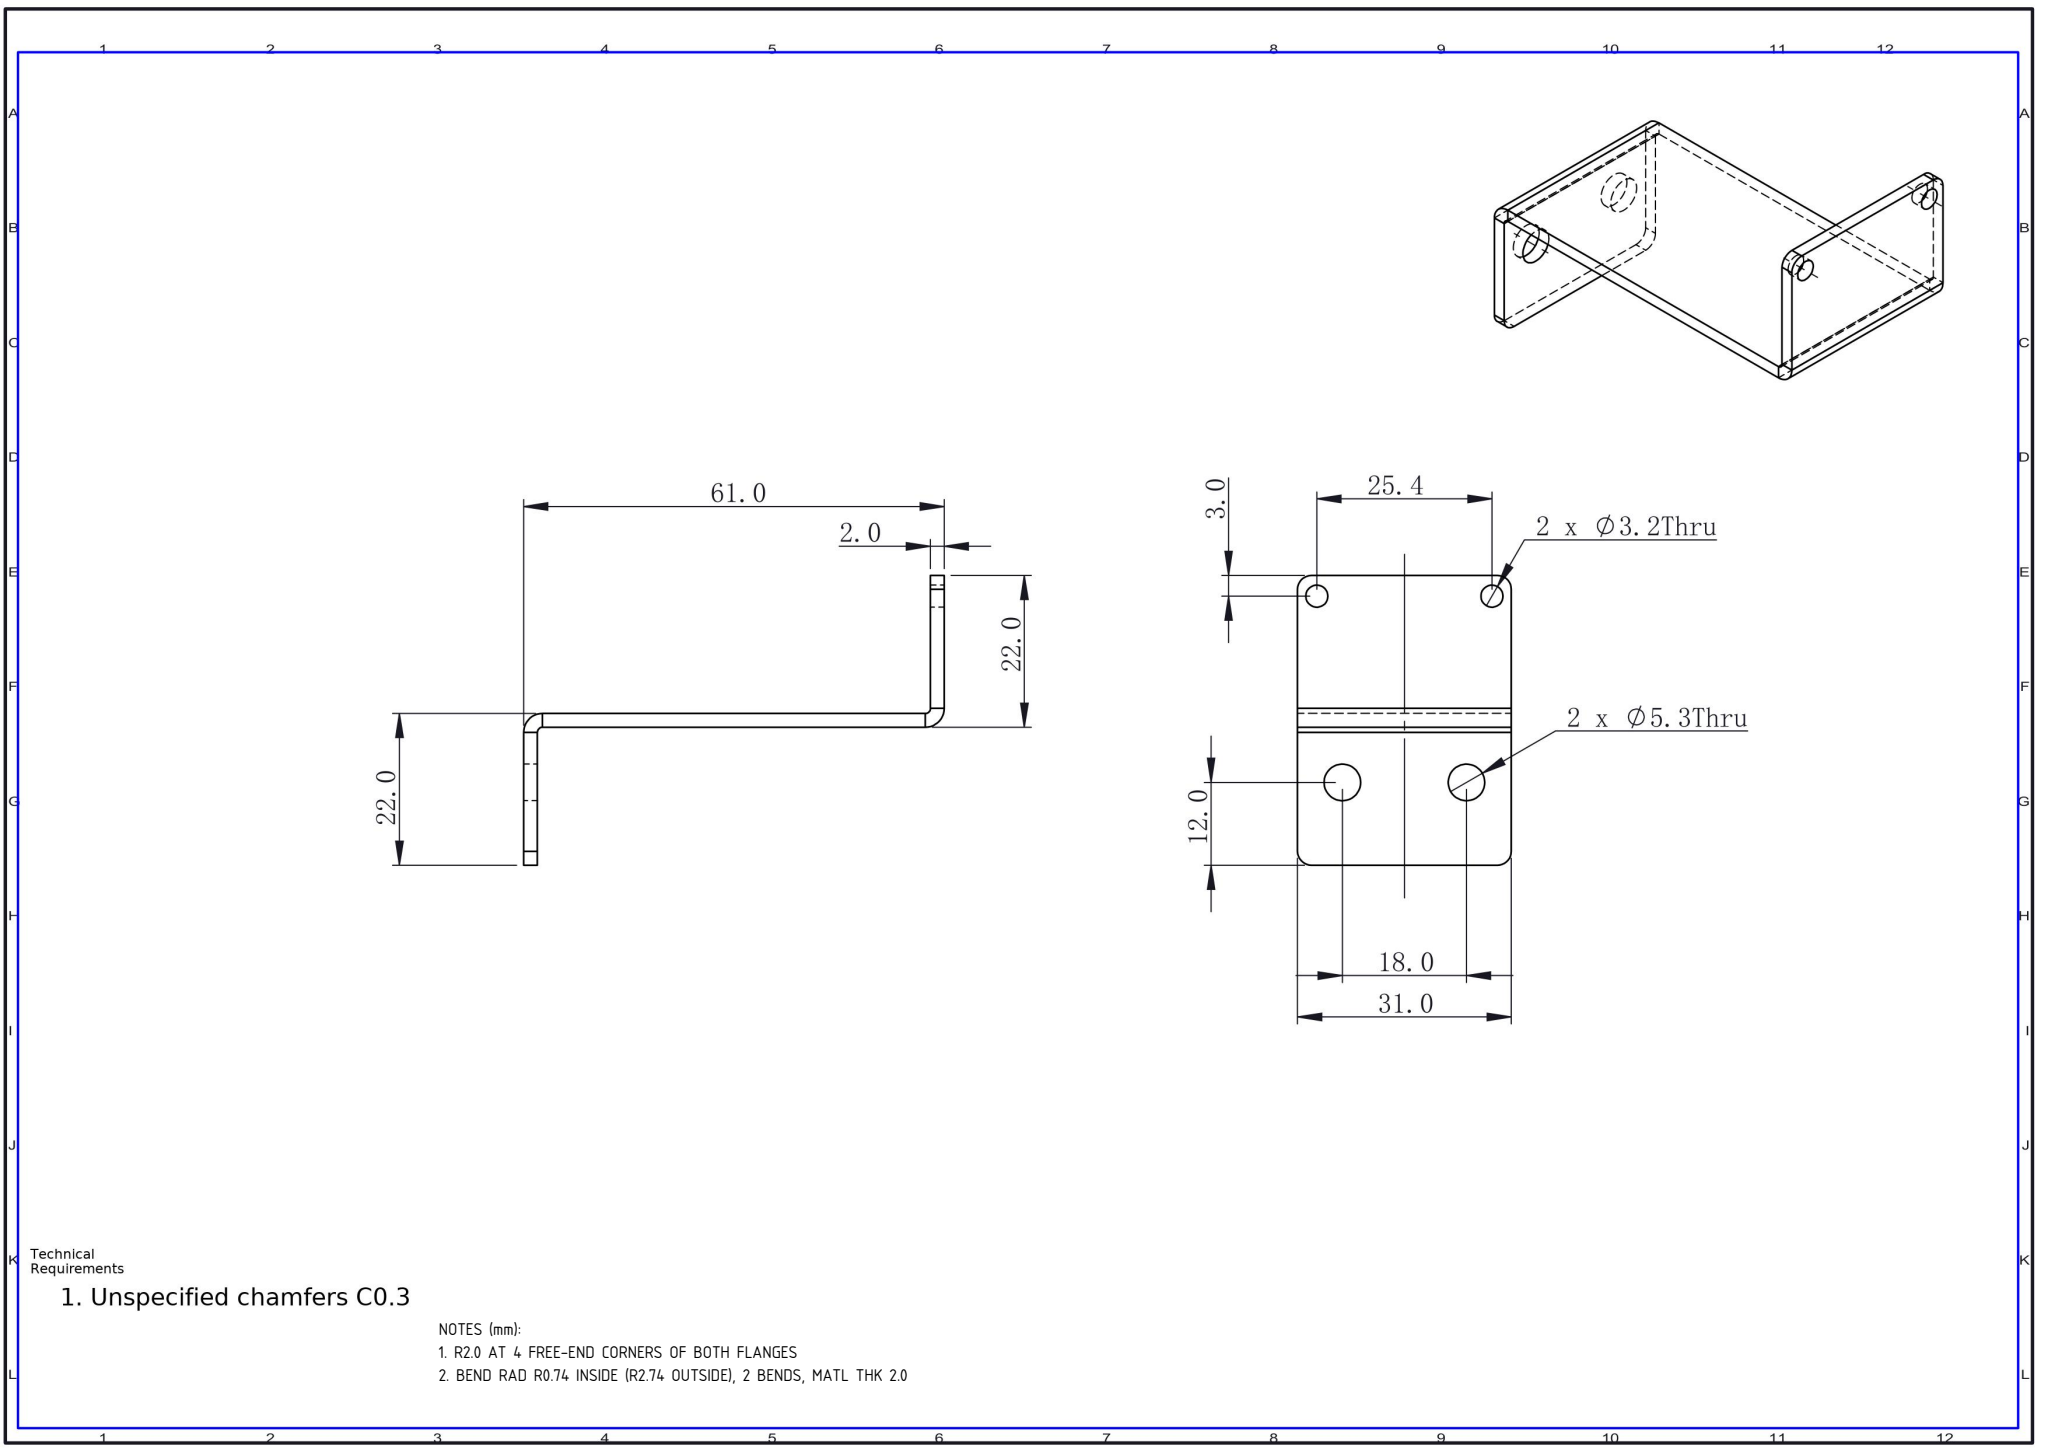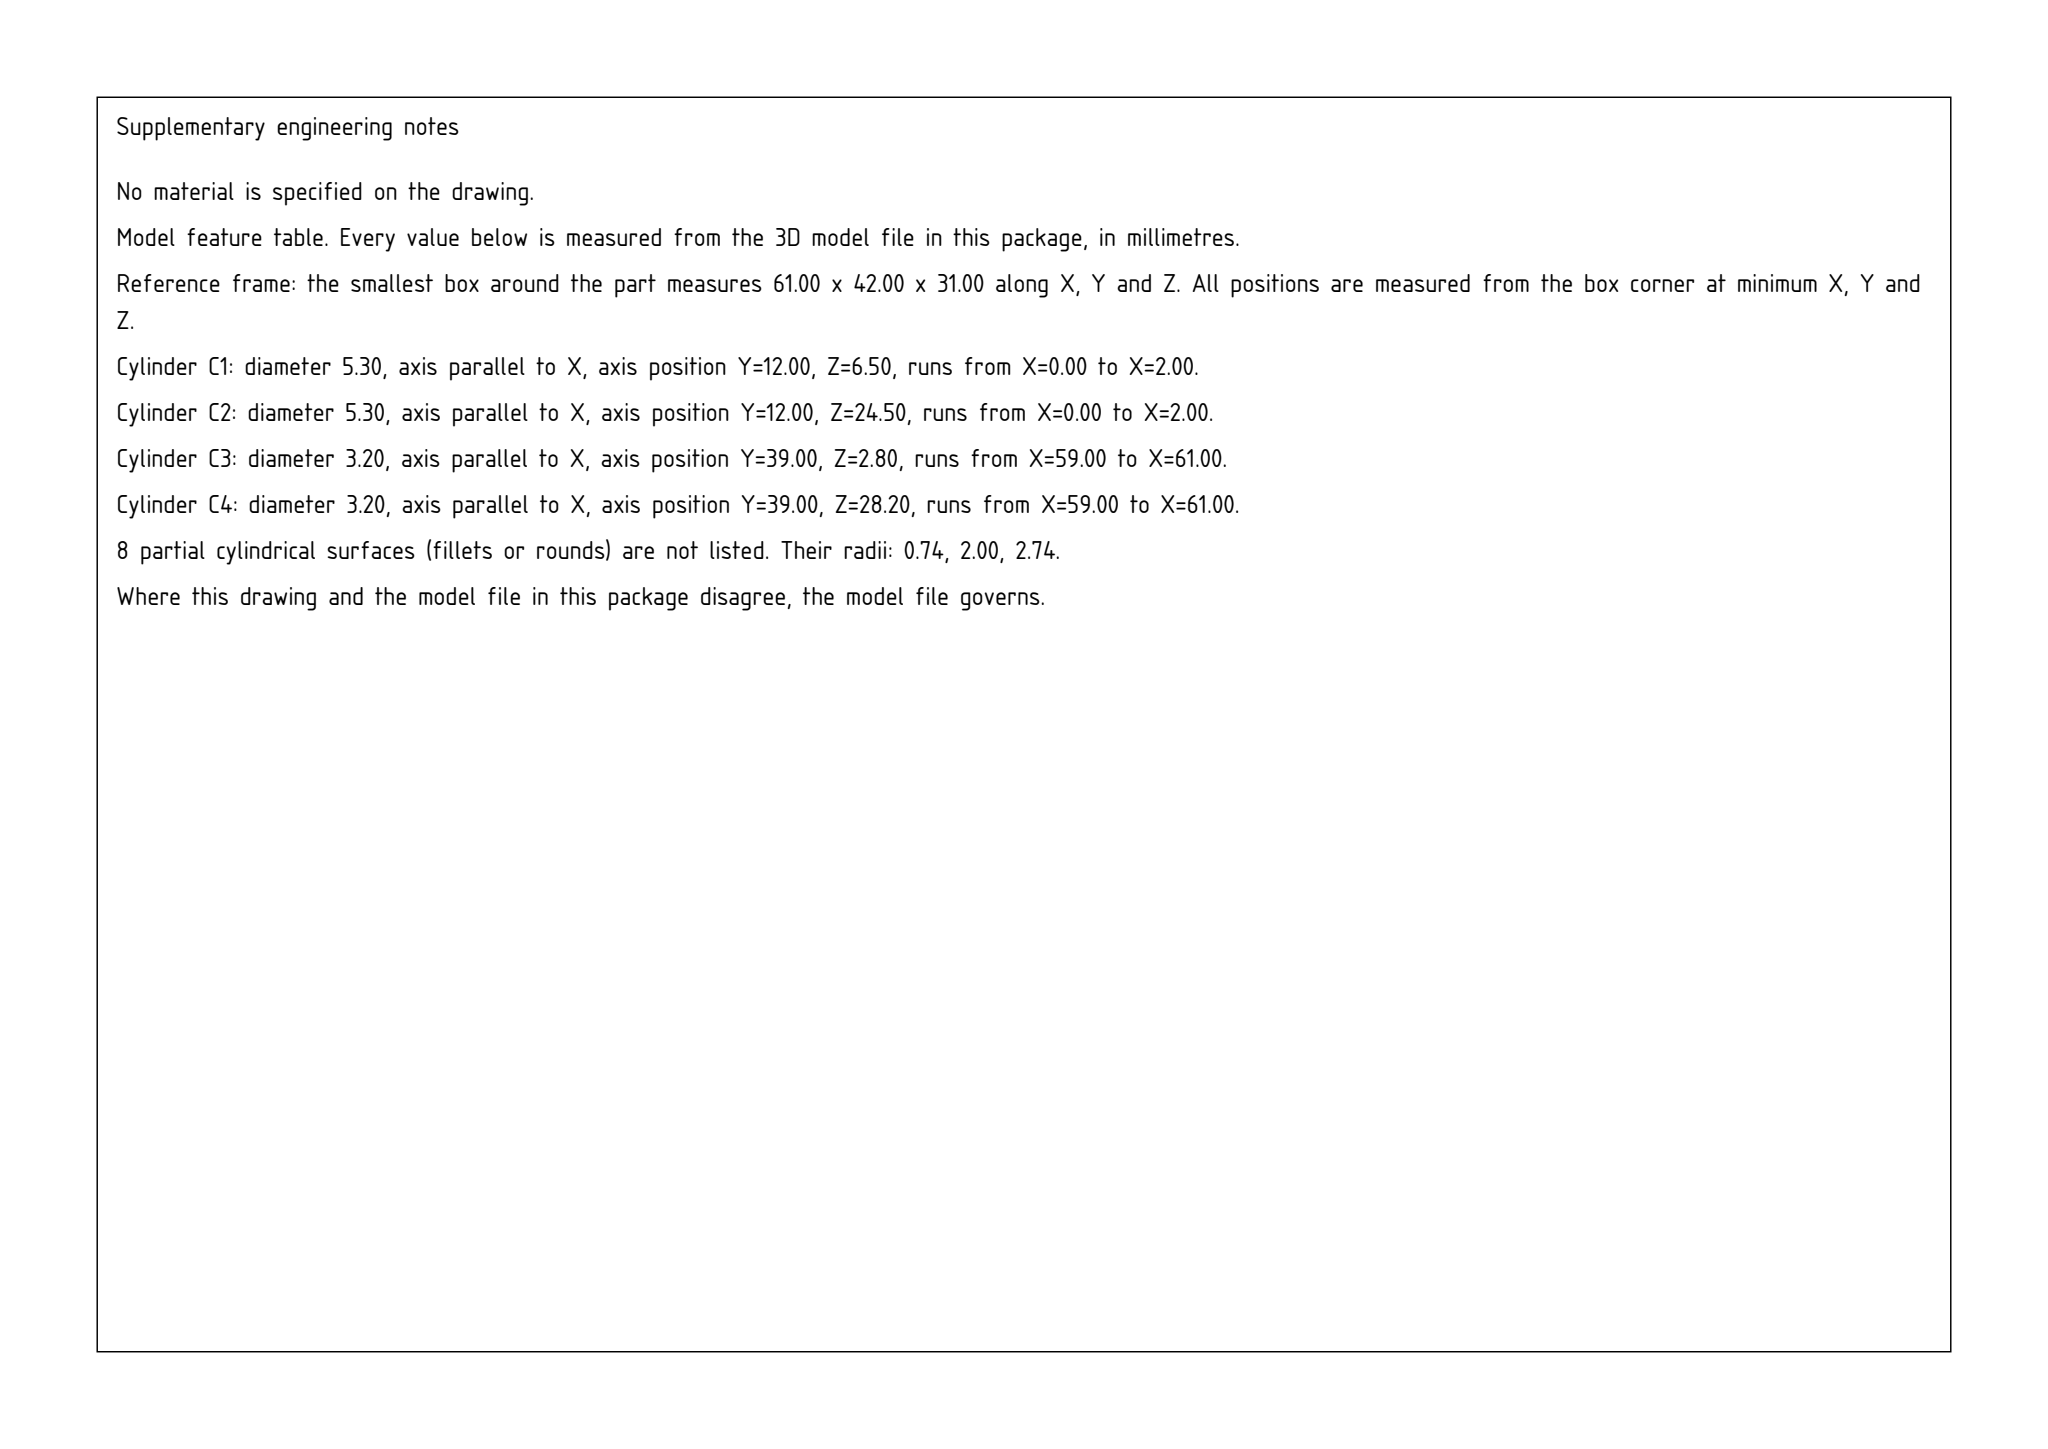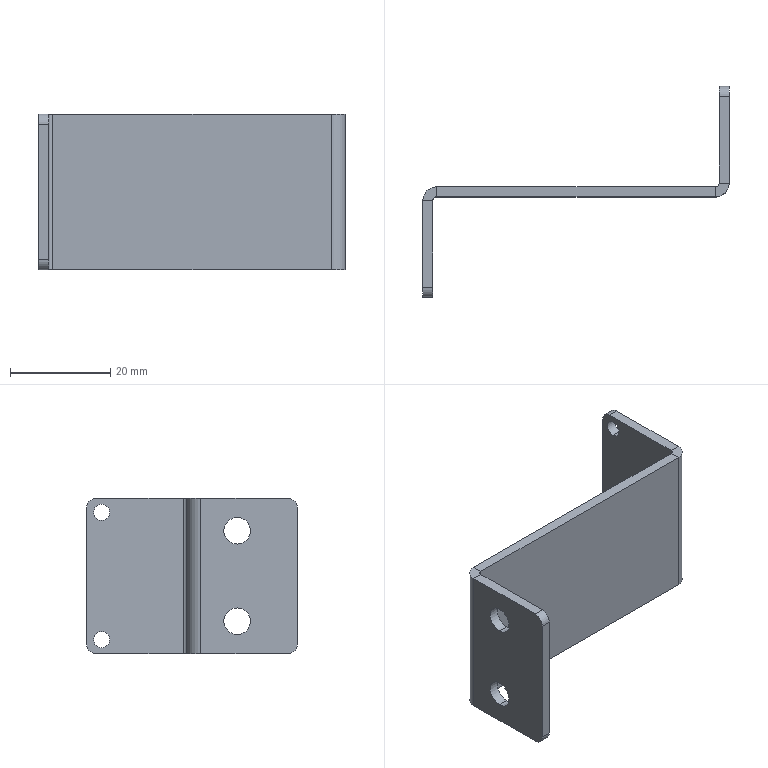Part | SolidWorks | mm | 1 solid | 34 faces | box 61 x 42 x 31 mm | volume 6042 mm3 | plane 18 | cylinder 16 | commonest cylinder face diameters 3.2 x4 5.3 x4 4 x4 1.473 x2 5.473 x2
Drawing notes:
R2.0 AT 4 FREE-END CORNERS OF BOTH FLANGES | from the solid: 4 x dia 4.0 cylinders, axis x, len 2.0, at (y,z)=(2,2),(2,29),(40,2),(40,29)
BEND RAD R0.74 INSIDE (R2.74 OUTSIDE), 2 BENDS, MATL THK 2.0 | from the solid: dia 1.473 & 5.473 z-axis cylinders at (2.74,19.26) and (58.26,22.74), len 31.0; planes x=0/2.0 and 59.0/61.0